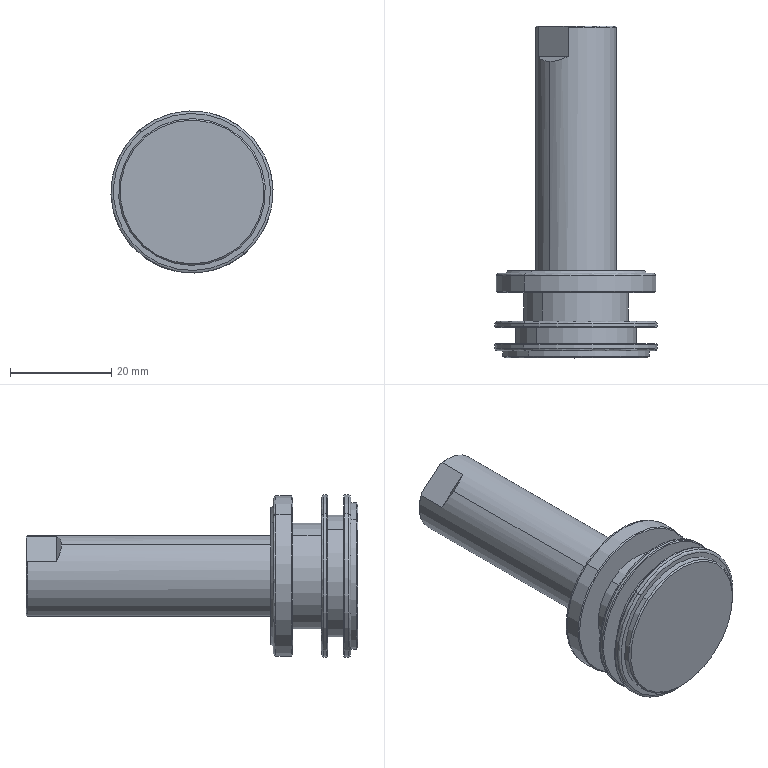Component | SolidWorks | SL021-113Q32x30S-2.SL41SM-1_SL021-113Q32x30S (1)-2.sl4prt-1 | 1 solid | 51 faces | volume 18733 mm3 | cylinder 16 | plane 13 | cone 12 | spline 10 | commonest cylinder face diameters 32 x4 16 x2 6.647 x2 31.6 x2 20.8 x2 24 x2 29 x2